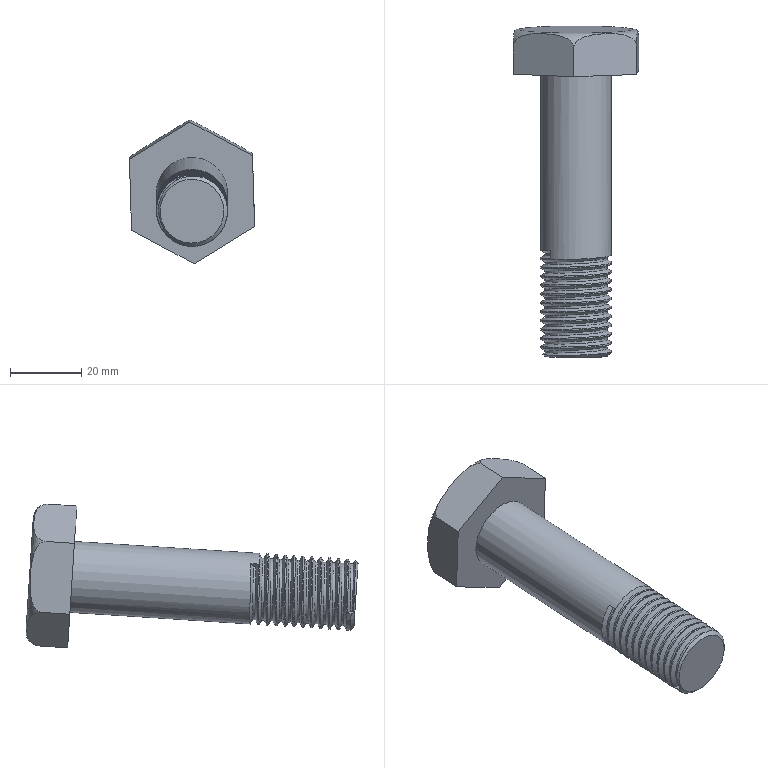Component | NX | CCJ-017 | 2 solids | 29 faces | volume 36161 mm3 | cylinder 13 | plane 12 | spline 2 | cone 1 | torus 1 | commonest cylinder face diameters 20 x12 17.5 x1